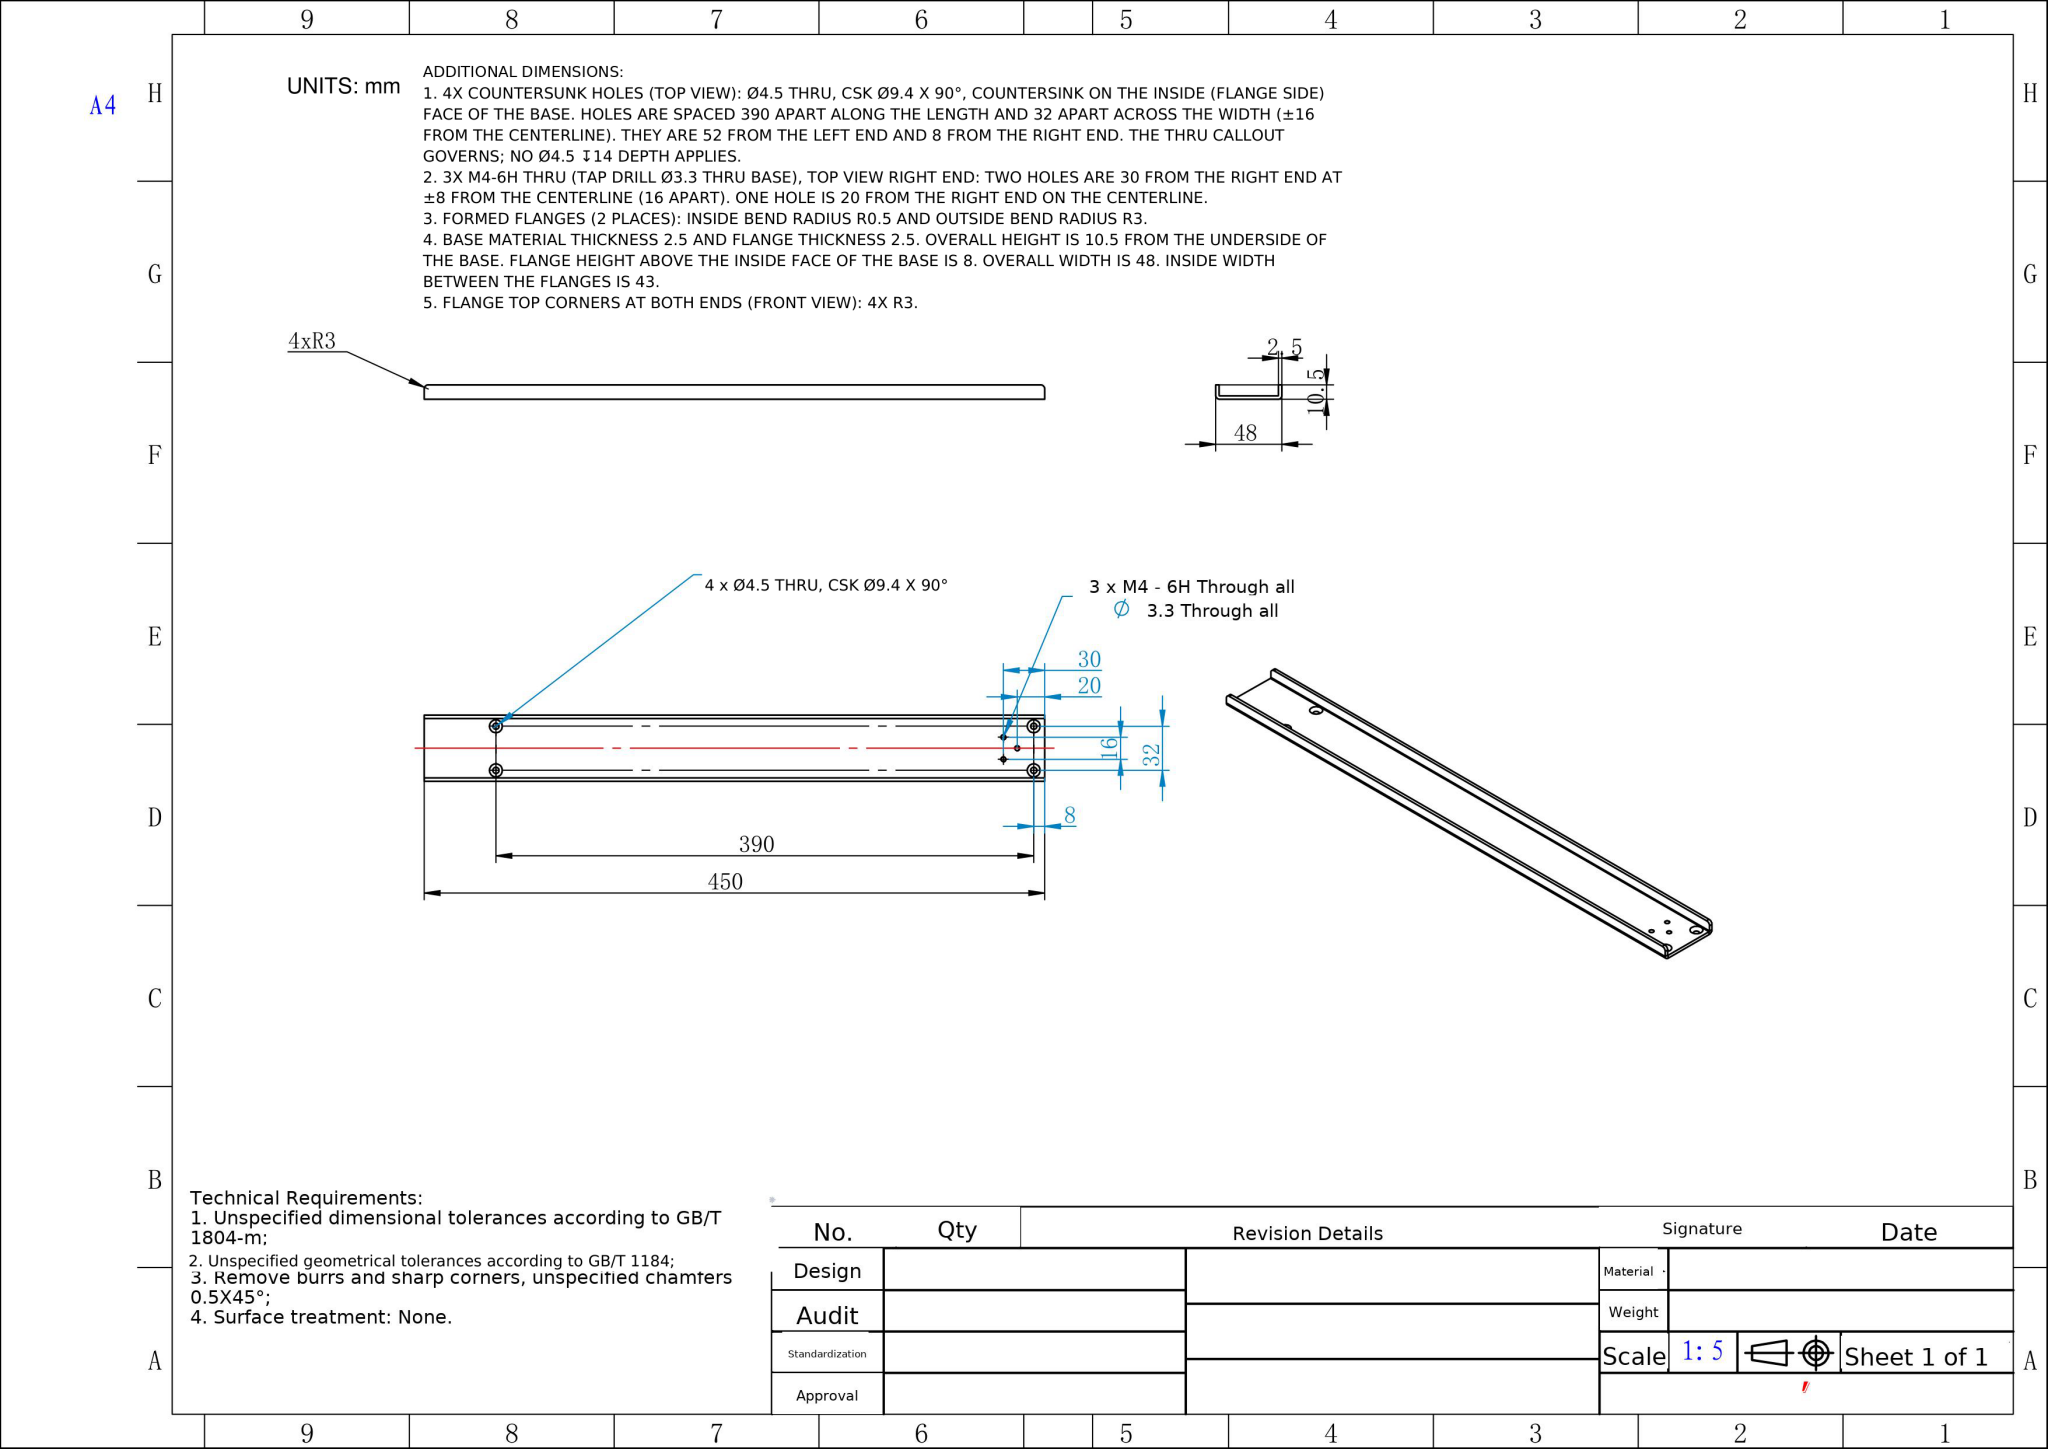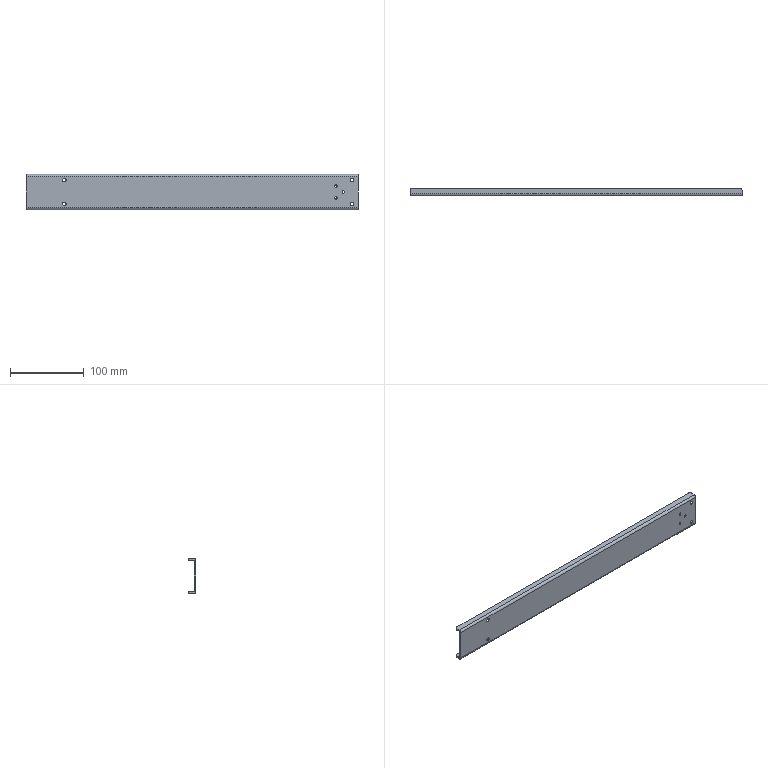Part | NX | mm | 1 solid | 48 faces | box 450 x 10.5 x 48 mm | volume 69836 mm3 | cylinder 22 | plane 18 | cone 8 | commonest cylinder face diameters 4.5 x8 3.3 x6 6 x6 1 x2